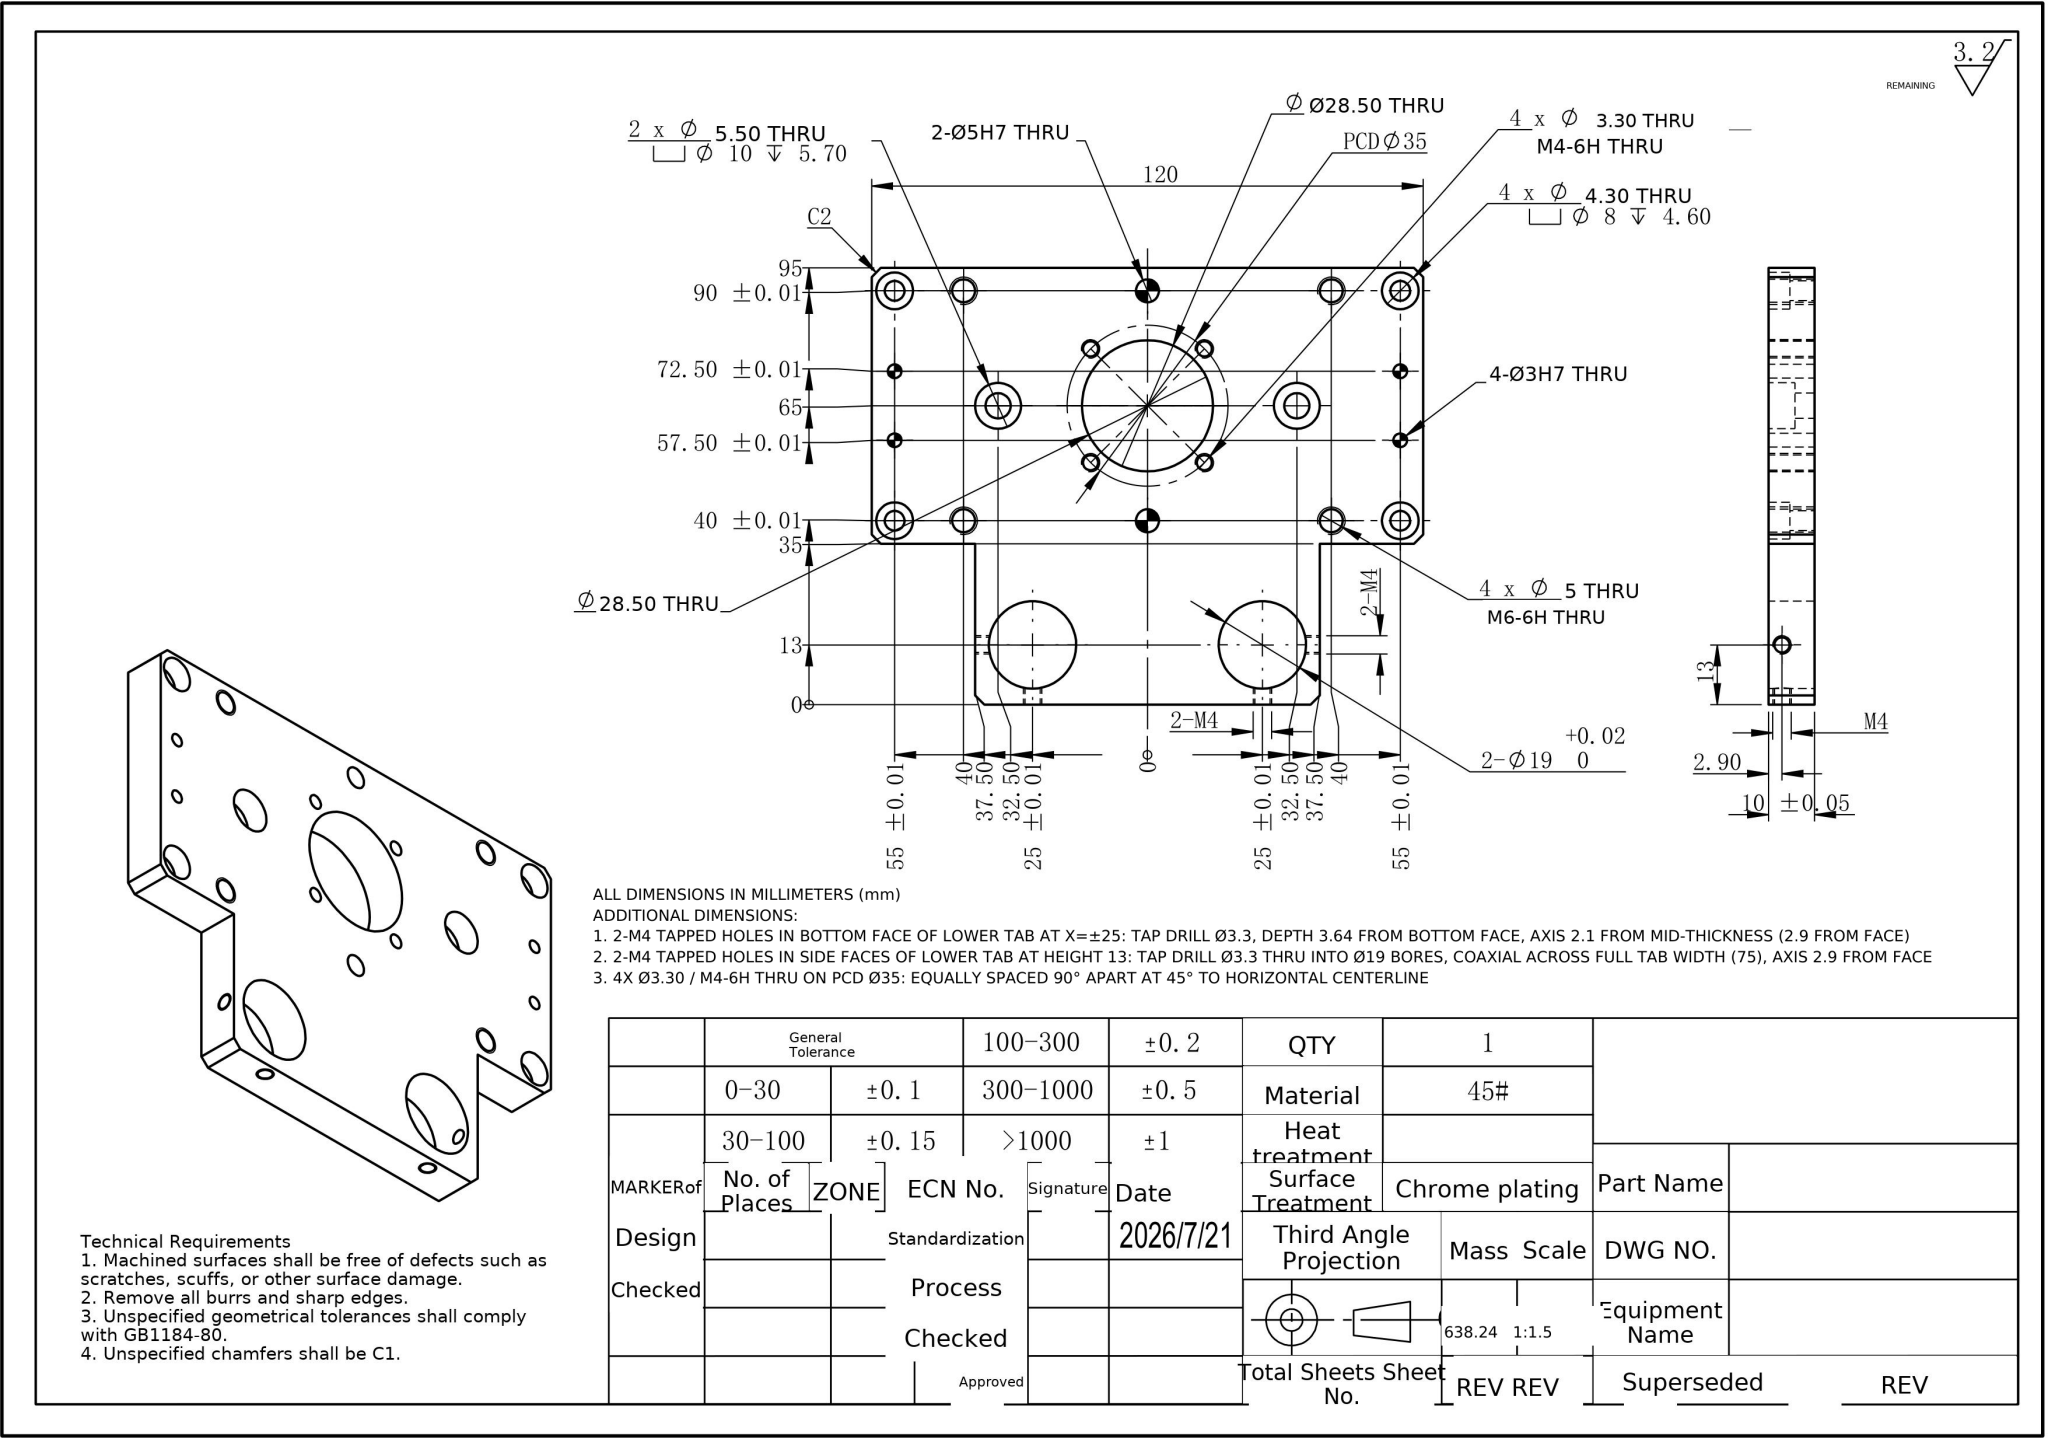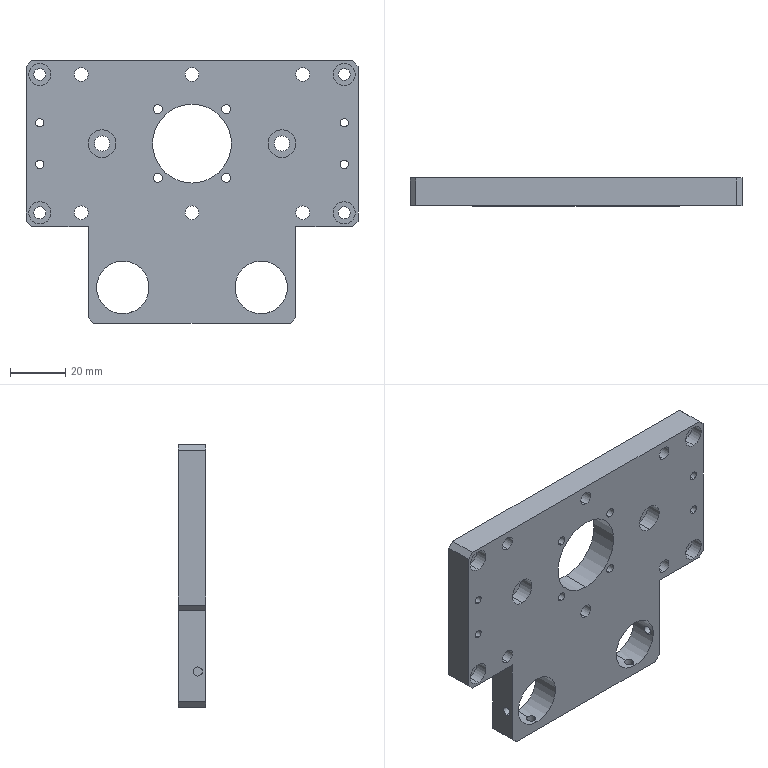Part | NX | mm | 1 solid | 88 faces | box 120 x 10 x 95 mm | volume 81826 mm3 | cylinder 66 | plane 22 | commonest cylinder face diameters 3.3 x16 5 x12 3 x8 8 x8 4.3 x8 19 x4 10 x4 5.5 x4